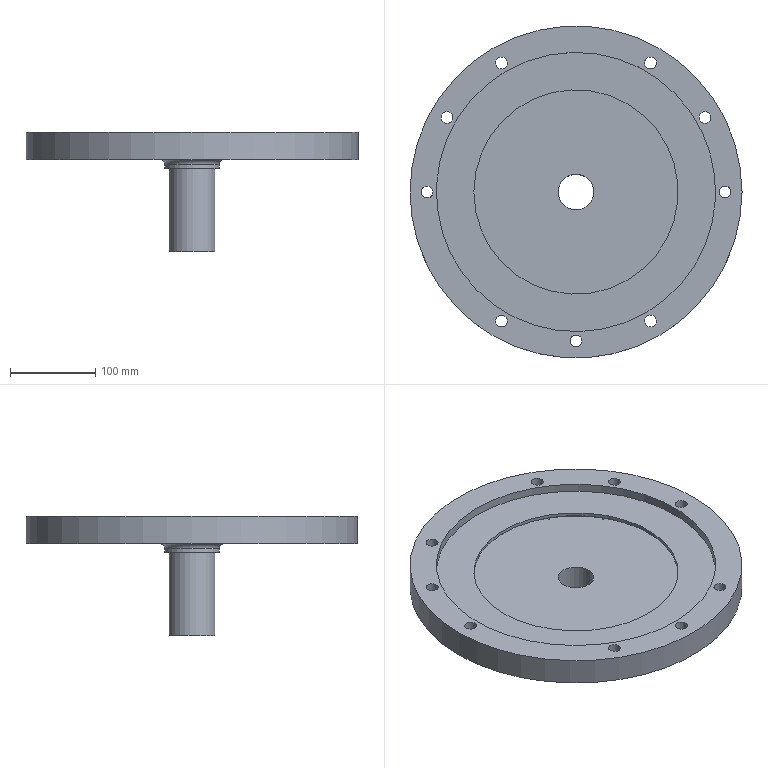Component | NX | DRIVEN_FLANGE | 1 solid | 66 faces | volume 2596868 mm3 | cylinder 40 | plane 19 | cone 6 | torus 1 | commonest cylinder face diameters 3 x12 14 x9 30 x6 11 x6 250 x1 42 x1 390 x1 54 x1